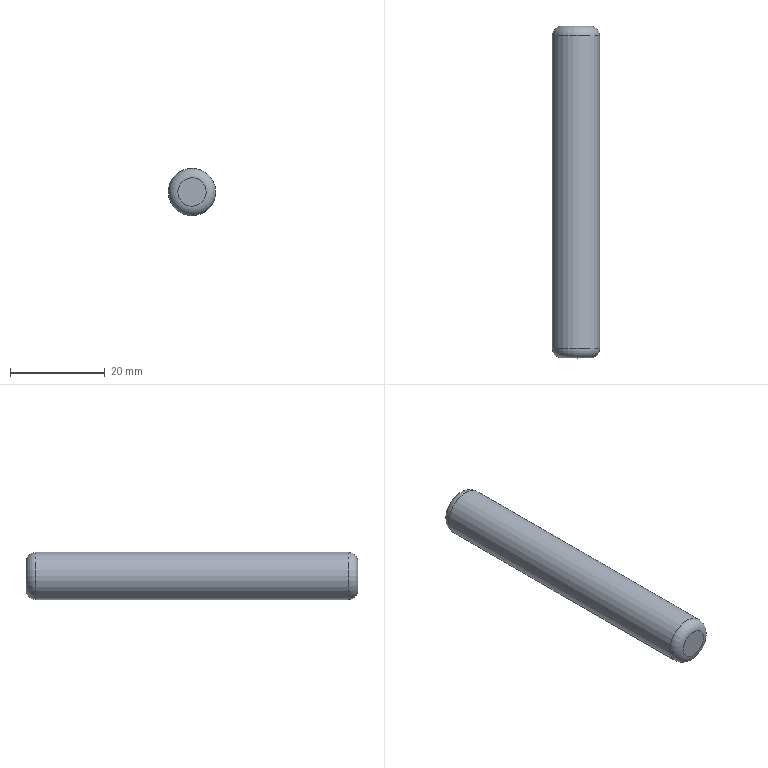Component | NX | CIBIK2 | 1 solid | 5 faces | box 10 x 70 x 10 mm | volume 5449 mm3 | plane 2 | torus 2 | cylinder 1 | commonest cylinder face diameters 10 x1
STEP:
#1=CARTESIAN_POINT('',(0.,0.,0.));
#2=DIRECTION('',(0.,0.,1.));
#3=DIRECTION('',(1.,0.,0.));
#4=AXIS2_PLACEMENT_3D('',#1,#2,#3);
#5=CARTESIAN_POINT('',(-1237.865,943.,230.062));
#6=VERTEX_POINT('',#5);
#7=CARTESIAN_POINT('',(-1239.575,943.,234.76));
#8=DIRECTION('',(0.,-1.,0.));
#9=DIRECTION('',(0.342,0.,-0.9397));
#10=AXIS2_PLACEMENT_3D('',#7,#8,#9);
#11=CIRCLE('',#10,5.);
#12=CARTESIAN_POINT('',(-1239.575,875.,234.76));
#13=DIRECTION('',(0.,1.,0.));
#14=DIRECTION('',(-0.342,0.,0.9397));
#15=AXIS2_PLACEMENT_3D('',#12,#13,#14);
#16=CYLINDRICAL_SURFACE('',#15,5.);
#17=CARTESIAN_POINT('',(9.425,68.));
#18=DIRECTION('',(-1.,0.));
#19=VECTOR('',#18,1.);
#20=LINE('',#17,#19);
#21=(GEOMETRIC_REPRESENTATION_CONTEXT(2)PARAMETRIC_REPRESENTATION_CONTEXT()REPRESENTATION_CONTEXT('',''));
#22=DEFINITIONAL_REPRESENTATION('',(#20),#21);
#23=PCURVE('',#16,#22);
#24=CARTESIAN_POINT('',(-1239.575,943.,234.76));
#25=DIRECTION('',(0.,-1.,0.));
#26=DIRECTION('',(0.342,0.,-0.9397));
#27=AXIS2_PLACEMENT_3D('',#24,#25,#26);
#28=TOROIDAL_SURFACE('',#27,3.,2.);
#29=CARTESIAN_POINT('',(0.,6.283));
#30=DIRECTION('',(1.,0.));
#31=VECTOR('',#30,1.);
#32=LINE('',#29,#31);
#33=(GEOMETRIC_REPRESENTATION_CONTEXT(2)PARAMETRIC_REPRESENTATION_CONTEXT()REPRESENTATION_CONTEXT('',''));
#34=DEFINITIONAL_REPRESENTATION('',(#32),#33);
#35=PCURVE('',#28,#34);
#36=SURFACE_CURVE('',#11,(#23,#35),.PCURVE_S1.);
#37=EDGE_CURVE('',#6,#6,#36,.T.);
#38=ORIENTED_EDGE('',*,*,#37,.T.);
#39=CARTESIAN_POINT('',(-1237.865,877.,230.062));
#40=VERTEX_POINT('',#39);
#41=CARTESIAN_POINT('',(-1237.865,877.,230.062));
#42=CARTESIAN_POINT('',(-1237.865,943.,230.062));
#43=B_SPLINE_CURVE_WITH_KNOTS('',1,(#41,#42),.UNSPECIFIED.,.F.,.F.,(2,2),(2.,68.),.PIECEWISE_BEZIER_KNOTS.);
#44=CARTESIAN_POINT('',(3.142,0.));
#45=DIRECTION('',(0.,1.));
#46=VECTOR('',#45,1.);
#47=LINE('',#44,#46);
#48=(GEOMETRIC_REPRESENTATION_CONTEXT(2)PARAMETRIC_REPRESENTATION_CONTEXT()REPRESENTATION_CONTEXT('',''));
#49=DEFINITIONAL_REPRESENTATION('',(#47),#48);
#50=PCURVE('',#16,#49);
#51=CARTESIAN_POINT('',(9.425,0.));
#52=DIRECTION('',(0.,1.));
#53=VECTOR('',#52,1.);
#54=LINE('',#51,#53);
#55=(GEOMETRIC_REPRESENTATION_CONTEXT(2)PARAMETRIC_REPRESENTATION_CONTEXT()REPRESENTATION_CONTEXT('',''));
#56=DEFINITIONAL_REPRESENTATION('',(#54),#55);
#57=PCURVE('',#16,#56);
#58=SEAM_CURVE('',#43,(#50,#57),.PCURVE_S1.);
#59=EDGE_CURVE('',#40,#6,#58,.T.);
#60=ORIENTED_EDGE('',*,*,#59,.F.);
#61=CARTESIAN_POINT('',(-1239.575,877.,234.76));
#62=DIRECTION('',(0.,1.,0.));
#63=DIRECTION('',(0.342,0.,-0.9397));
#64=AXIS2_PLACEMENT_3D('',#61,#62,#63);
#65=CIRCLE('',#64,5.);
#66=CARTESIAN_POINT('',(3.142,2.));
#67=DIRECTION('',(1.,0.));
#68=VECTOR('',#67,1.);
#69=LINE('',#66,#68);
#70=(GEOMETRIC_REPRESENTATION_CONTEXT(2)PARAMETRIC_REPRESENTATION_CONTEXT()REPRESENTATION_CONTEXT('',''));
#71=DEFINITIONAL_REPRESENTATION('',(#69),#70);
#72=PCURVE('',#16,#71);
#73=CARTESIAN_POINT('',(-1239.575,877.,234.76));
#74=DIRECTION('',(0.,-1.,0.));
#75=DIRECTION('',(0.342,0.,-0.9397));
#76=AXIS2_PLACEMENT_3D('',#73,#74,#75);
#77=TOROIDAL_SURFACE('',#76,3.,2.);
#78=CARTESIAN_POINT('',(6.283,6.283));
#79=DIRECTION('',(-1.,0.));
#80=VECTOR('',#79,1.);
#81=LINE('',#78,#80);
#82=(GEOMETRIC_REPRESENTATION_CONTEXT(2)PARAMETRIC_REPRESENTATION_CONTEXT()REPRESENTATION_CONTEXT('',''));
#83=DEFINITIONAL_REPRESENTATION('',(#81),#82);
#84=PCURVE('',#77,#83);
#85=SURFACE_CURVE('',#65,(#72,#84),.PCURVE_S1.);
#86=EDGE_CURVE('',#40,#40,#85,.T.);
#87=ORIENTED_EDGE('',*,*,#86,.T.);
#88=ORIENTED_EDGE('',*,*,#59,.T.);
#89=EDGE_LOOP('',(#38,#60,#87,#88));
#90=FACE_BOUND('',#89,.T.);
#91=ADVANCED_FACE('',(#90),#16,.T.);
#92=CARTESIAN_POINT('',(-1238.549,875.,231.941));
#93=VERTEX_POINT('',#92);
#94=CARTESIAN_POINT('',(-1239.575,875.,234.76));
#95=DIRECTION('',(0.,-1.,0.));
#96=DIRECTION('',(0.342,0.,-0.9397));
#97=AXIS2_PLACEMENT_3D('',#94,#95,#96);
#98=CIRCLE('',#97,3.);
#99=CARTESIAN_POINT('',(-1239.575,875.,234.76));
#100=DIRECTION('',(0.,-1.,0.));
#101=DIRECTION('',(0.342,0.,-0.9397));
#102=AXIS2_PLACEMENT_3D('',#99,#100,#101);
#103=PLANE('',#102);
#104=CARTESIAN_POINT('',(0.,0.));
#105=DIRECTION('',(1.,-0.));
#106=AXIS2_PLACEMENT_2D('',#104,#105);
#107=CIRCLE('',#106,3.);
#108=(GEOMETRIC_REPRESENTATION_CONTEXT(2)PARAMETRIC_REPRESENTATION_CONTEXT()REPRESENTATION_CONTEXT('',''));
#109=DEFINITIONAL_REPRESENTATION('',(#107),#108);
#110=PCURVE('',#103,#109);
#111=CARTESIAN_POINT('',(0.,7.854));
#112=DIRECTION('',(1.,0.));
#113=VECTOR('',#112,1.);
#114=LINE('',#111,#113);
#115=(GEOMETRIC_REPRESENTATION_CONTEXT(2)PARAMETRIC_REPRESENTATION_CONTEXT()REPRESENTATION_CONTEXT('',''));
#116=DEFINITIONAL_REPRESENTATION('',(#114),#115);
#117=PCURVE('',#77,#116);
#118=SURFACE_CURVE('',#98,(#110,#117),.PCURVE_S1.);
#119=EDGE_CURVE('',#93,#93,#118,.T.);
#120=ORIENTED_EDGE('',*,*,#119,.T.);
#121=EDGE_LOOP('',(#120));
#122=FACE_BOUND('',#121,.T.);
#123=ADVANCED_FACE('',(#122),#103,.T.);
#124=CARTESIAN_POINT('',(-1238.549,945.,231.941));
#125=VERTEX_POINT('',#124);
#126=CARTESIAN_POINT('',(-1239.575,945.,234.76));
#127=DIRECTION('',(0.,1.,0.));
#128=DIRECTION('',(0.342,0.,-0.9397));
#129=AXIS2_PLACEMENT_3D('',#126,#127,#128);
#130=CIRCLE('',#129,3.);
#131=CARTESIAN_POINT('',(-1239.575,945.,234.76));
#132=DIRECTION('',(0.,-1.,0.));
#133=DIRECTION('',(0.342,0.,-0.9397));
#134=AXIS2_PLACEMENT_3D('',#131,#132,#133);
#135=PLANE('',#134);
#136=CARTESIAN_POINT('',(3.,-0.));
#137=CARTESIAN_POINT('',(3.,-5.196));
#138=CARTESIAN_POINT('',(-1.5,-2.598));
#139=CARTESIAN_POINT('',(-6.,0.));
#140=CARTESIAN_POINT('',(-1.5,2.598));
#141=CARTESIAN_POINT('',(3.,5.196));
#142=CARTESIAN_POINT('',(3.,-0.));
#143=(BOUNDED_CURVE()B_SPLINE_CURVE(2,(#136,#137,#138,#139,#140,#141,#142),.UNSPECIFIED.,.T.,.F.)B_SPLINE_CURVE_WITH_KNOTS((1,2,2,2,2,1),(-2.094,0.,2.094,4.189,6.283,8.378),.UNSPECIFIED.)CURVE()GEOMETRIC_REPRESENTATION_ITEM()RATIONAL_B_SPLINE_CURVE((1.,0.5,1.,0.5,1.,0.5,1.))REPRESENTATION_ITEM(''));
#144=(GEOMETRIC_REPRESENTATION_CONTEXT(2)PARAMETRIC_REPRESENTATION_CONTEXT()REPRESENTATION_CONTEXT('',''));
#145=DEFINITIONAL_REPRESENTATION('',(#143),#144);
#146=PCURVE('',#135,#145);
#147=CARTESIAN_POINT('',(6.283,4.712));
#148=DIRECTION('',(-1.,0.));
#149=VECTOR('',#148,1.);
#150=LINE('',#147,#149);
#151=(GEOMETRIC_REPRESENTATION_CONTEXT(2)PARAMETRIC_REPRESENTATION_CONTEXT()REPRESENTATION_CONTEXT('',''));
#152=DEFINITIONAL_REPRESENTATION('',(#150),#151);
#153=PCURVE('',#28,#152);
#154=SURFACE_CURVE('',#130,(#146,#153),.PCURVE_S1.);
#155=EDGE_CURVE('',#125,#125,#154,.T.);
#156=ORIENTED_EDGE('',*,*,#155,.T.);
#157=EDGE_LOOP('',(#156));
#158=FACE_BOUND('',#157,.T.);
#159=ADVANCED_FACE('',(#158),#135,.F.);
#160=ORIENTED_EDGE('',*,*,#155,.F.);
#161=CARTESIAN_POINT('',(-1238.549,945.,231.941));
#162=CARTESIAN_POINT('',(-1238.366,945.,231.439));
#163=CARTESIAN_POINT('',(-1238.188,944.83,230.949));
#164=CARTESIAN_POINT('',(-1238.034,944.504,230.528));
#165=CARTESIAN_POINT('',(-1237.923,944.055,230.221));
#166=CARTESIAN_POINT('',(-1237.865,943.535,230.062));
#167=CARTESIAN_POINT('',(-1237.865,943.,230.062));
#168=(BOUNDED_CURVE()B_SPLINE_CURVE(6,(#161,#162,#163,#164,#165,#166,#167),.UNSPECIFIED.,.F.,.F.)B_SPLINE_CURVE_WITH_KNOTS((7,7),(4.712,6.283),.PIECEWISE_BEZIER_KNOTS.)CURVE()GEOMETRIC_REPRESENTATION_ITEM()RATIONAL_B_SPLINE_CURVE((1.031,1.01,0.9979,0.994,0.9979,1.01,1.031))REPRESENTATION_ITEM(''));
#169=CARTESIAN_POINT('',(6.283,0.));
#170=DIRECTION('',(0.,1.));
#171=VECTOR('',#170,1.);
#172=LINE('',#169,#171);
#173=(GEOMETRIC_REPRESENTATION_CONTEXT(2)PARAMETRIC_REPRESENTATION_CONTEXT()REPRESENTATION_CONTEXT('',''));
#174=DEFINITIONAL_REPRESENTATION('',(#172),#173);
#175=PCURVE('',#28,#174);
#176=CARTESIAN_POINT('',(0.,0.));
#177=DIRECTION('',(0.,1.));
#178=VECTOR('',#177,1.);
#179=LINE('',#176,#178);
#180=(GEOMETRIC_REPRESENTATION_CONTEXT(2)PARAMETRIC_REPRESENTATION_CONTEXT()REPRESENTATION_CONTEXT('',''));
#181=DEFINITIONAL_REPRESENTATION('',(#179),#180);
#182=PCURVE('',#28,#181);
#183=SEAM_CURVE('',#168,(#175,#182),.PCURVE_S1.);
#184=EDGE_CURVE('',#125,#6,#183,.T.);
#185=ORIENTED_EDGE('',*,*,#184,.T.);
#186=ORIENTED_EDGE('',*,*,#37,.F.);
#187=ORIENTED_EDGE('',*,*,#184,.F.);
#188=EDGE_LOOP('',(#160,#185,#186,#187));
#189=FACE_BOUND('',#188,.T.);
#190=ADVANCED_FACE('',(#189),#28,.T.);
#191=ORIENTED_EDGE('',*,*,#86,.F.);
#192=CARTESIAN_POINT('',(-1237.865,877.,230.062));
#193=CARTESIAN_POINT('',(-1237.865,876.465,230.062));
#194=CARTESIAN_POINT('',(-1237.923,875.945,230.221));
#195=CARTESIAN_POINT('',(-1238.034,875.496,230.528));
#196=CARTESIAN_POINT('',(-1238.188,875.17,230.949));
#197=CARTESIAN_POINT('',(-1238.366,875.,231.439));
#198=CARTESIAN_POINT('',(-1238.549,875.,231.941));
#199=(BOUNDED_CURVE()B_SPLINE_CURVE(6,(#192,#193,#194,#195,#196,#197,#198),.UNSPECIFIED.,.F.,.F.)B_SPLINE_CURVE_WITH_KNOTS((7,7),(0.,1.571),.PIECEWISE_BEZIER_KNOTS.)CURVE()GEOMETRIC_REPRESENTATION_ITEM()RATIONAL_B_SPLINE_CURVE((1.031,1.01,0.9979,0.994,0.9979,1.01,1.031))REPRESENTATION_ITEM(''));
#200=CARTESIAN_POINT('',(6.283,6.283));
#201=DIRECTION('',(0.,1.));
#202=VECTOR('',#201,1.);
#203=LINE('',#200,#202);
#204=(GEOMETRIC_REPRESENTATION_CONTEXT(2)PARAMETRIC_REPRESENTATION_CONTEXT()REPRESENTATION_CONTEXT('',''));
#205=DEFINITIONAL_REPRESENTATION('',(#203),#204);
#206=PCURVE('',#77,#205);
#207=CARTESIAN_POINT('',(0.,6.283));
#208=DIRECTION('',(0.,1.));
#209=VECTOR('',#208,1.);
#210=LINE('',#207,#209);
#211=(GEOMETRIC_REPRESENTATION_CONTEXT(2)PARAMETRIC_REPRESENTATION_CONTEXT()REPRESENTATION_CONTEXT('',''));
#212=DEFINITIONAL_REPRESENTATION('',(#210),#211);
#213=PCURVE('',#77,#212);
#214=SEAM_CURVE('',#199,(#206,#213),.PCURVE_S1.);
#215=EDGE_CURVE('',#40,#93,#214,.T.);
#216=ORIENTED_EDGE('',*,*,#215,.T.);
#217=ORIENTED_EDGE('',*,*,#119,.F.);
#218=ORIENTED_EDGE('',*,*,#215,.F.);
#219=EDGE_LOOP('',(#191,#216,#217,#218));
#220=FACE_BOUND('',#219,.T.);
#221=ADVANCED_FACE('',(#220),#77,.T.);
#222=CLOSED_SHELL('',(#91,#123,#159,#190,#221));
#223=MANIFOLD_SOLID_BREP('',#222);
#224=(LENGTH_UNIT()NAMED_UNIT(*)SI_UNIT(.MILLI.,.METRE.));
#225=UNCERTAINTY_MEASURE_WITH_UNIT(LENGTH_MEASURE(0.00001),#224,'','');
#226=(NAMED_UNIT(*)PLANE_ANGLE_UNIT()SI_UNIT($,.RADIAN.));
#227=(NAMED_UNIT(*)SI_UNIT($,.STERADIAN.)SOLID_ANGLE_UNIT());
#228=(GEOMETRIC_REPRESENTATION_CONTEXT(3)GLOBAL_UNCERTAINTY_ASSIGNED_CONTEXT((#225))GLOBAL_UNIT_ASSIGNED_CONTEXT((#224,#226,#227))REPRESENTATION_CONTEXT('',''));
#229=ADVANCED_BREP_SHAPE_REPRESENTATION('',(#4,#223),#228);